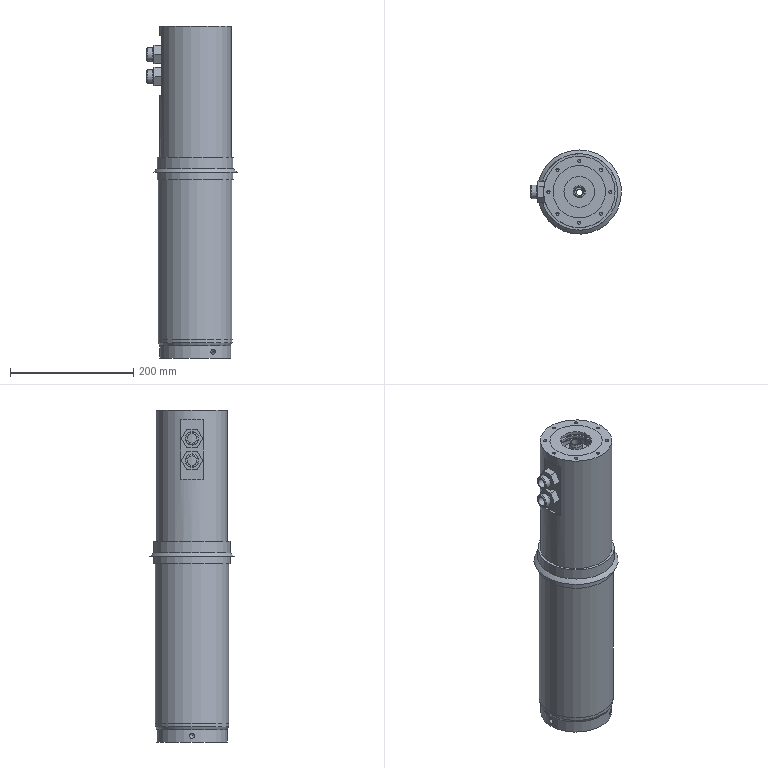Assembly | NX | mm | 19 component files | 19 solids | 298 faces | box 147.25 x 136.5 x 538 mm | volume 4269559 mm3 | cylinder 121 | plane 108 | cone 54 | sphere 9 | torus 5 | spline 1 | commonest cylinder face diameters 5 x26 20 x8 85 x8 30 x5 45 x5 24.6 x4 95 x4 22 x4
Bill of materials:
CH3404.8-4 | 1 |  | Spool-shaped body that turns around one axis. It has three full-diameter flange bands with recessed necks between them, a counterbored top opening with internal ridges, and a small central through-hole.
CH3404.8-5 | 9 |  | Solid plain cylinder, roughly twice as long as its diameter. One end is a flat circular face with a small chamfered or rounded edge. The other end is slightly domed or crowned, with a rounded edge.
CH3404.8.2-1 | 1 |  | Long thin-walled tube with a large bore. The upper section has a slightly smaller outer diameter, a narrow raised collar band sits about a third of the way up, and eight small holes or dimples are evenly spaced on the top end face.
CH3404.8-2 | 1 |  | Thick-walled cylindrical sleeve with a chamfered top outer edge and a stepped bore with internal ridges near the top. It has three small axial holes in the top face and small radial holes through the side wall in two rows along the height.
CH3404.8-1 | 1 |  | Stepped cylindrical cup-shaped housing. From the bottom up it has a base band with radial holes, a wider chamfered flange, a relief groove, an intermediate-diameter band, and an upper cylinder with two grooves near the top. Inside, a central boss has a small through-bore.
CH3404.8.2 | 1 |  | Thin flat ring with a large inner diameter and a narrow radial width. In side view its cross-section is a trapezoid, which suggests a beveled or conical edge.
CH3404.8-6 | 2 |  | Symmetric hollow fitting-like body with a central hexagonal section and two coaxial cylindrical ends. The ends have chamfered edges and are joined to the hex by reduced-diameter necks. There is a through-bore.
CH3404.8.1-2 | 1 |  | Long slender thin-walled tube with a short reduced-diameter section at one end.
CH3404.8.1-1 | 1 |  | Short thick-walled cylindrical bushing or sleeve with a stepped bore: a counterbore from one end ends at an internal shoulder. One outer end edge is chamfered.
CH3404.8-3 | 1 |  | Very slender thin-walled tube with short reduced-diameter sections at both ends.
Mates:
1. touch align | CH3404_8_1-2 1 face | CH3404_8_1-1 1 face
2. touch align | CH3404_8_1-2 1 face | CH3404_8_1-1 1 face
3. fix | CH3404_8_2-1 1 component
4. fix | CH3404_8-1 1 component
5. touch align | CH3404_8-2 1 face | CH3404_8-1 1 face
6. touch align | CH3404_8-2 1 face | assembly datumplane
7. touch align | CH3404_8-3 1 face | CH3404_8-1 1 face
8. touch align | CH3404_8-3 1 face | CH3404_8-1 1 face
9. touch align | CH3404_8_1 1 face | CH3404_8-1 1 face
10. touch align | CH3404_8_1 1 face | CH3404_8-2 1 face
11. touch align | CH3404_8_2 1 face | CH3404_8-1 1 face
12. touch align | CH3404_8_2 1 face | CH3404_8-1 1 face
13. touch align | CH3404_8-4 1 face | CH3404_8_2 1 face
14. parallel | CH3404_8_2 1 datumplane | assembly datumplane
15. parallel | CH3404_8-4 1 datumplane | assembly datumplane
16. touch align | CH3404_8-5 9 face | CH3404_8-2 1 face
17. touch align | CH3404_8-5 8 face | CH3404_8-2 1 face
18. touch align | CH3404_8-5 7 face | CH3404_8-2 1 face
19. touch align | CH3404_8-5 6 face | CH3404_8-2 1 face
20. touch align | CH3404_8-5 5 face | CH3404_8-2 1 face
21. touch align | CH3404_8-5 9 face | CH3404_8-1 1 face
22. touch align | CH3404_8-5 7 face | CH3404_8-1 1 face
23. touch align | CH3404_8-5 8 face | CH3404_8-1 1 face
24. touch align | CH3404_8-5 6 face | CH3404_8-1 1 face
25. touch align | CH3404_8-5 5 face | CH3404_8-1 1 face
26. touch align | CH3404_8-5 4 face | CH3404_8-2 1 face
27. touch align | CH3404_8-5 3 face | CH3404_8-2 1 face
28. touch align | CH3404_8-5 2 face | CH3404_8-2 1 face
29. touch align | CH3404_8-5 1 face | CH3404_8-2 1 face
30. touch align | CH3404_8-5 2 face | CH3404_8-1 1 face
31. touch align | CH3404_8-5 4 face | CH3404_8-1 1 face
32. touch align | CH3404_8-5 1 face | CH3404_8-1 1 face
33. touch align | CH3404_8-5 3 face | CH3404_8-1 1 face
34. touch align | CH3404_8-6 2 face | CH3404_8_2 1
35. touch align | CH3404_8-6 1 face | CH3404_8_2 1
36. touch align | CH3404_8-6 2 face | CH3404_8_2 1 face
37. touch align | CH3404_8-6 1 face | CH3404_8_2 1 face